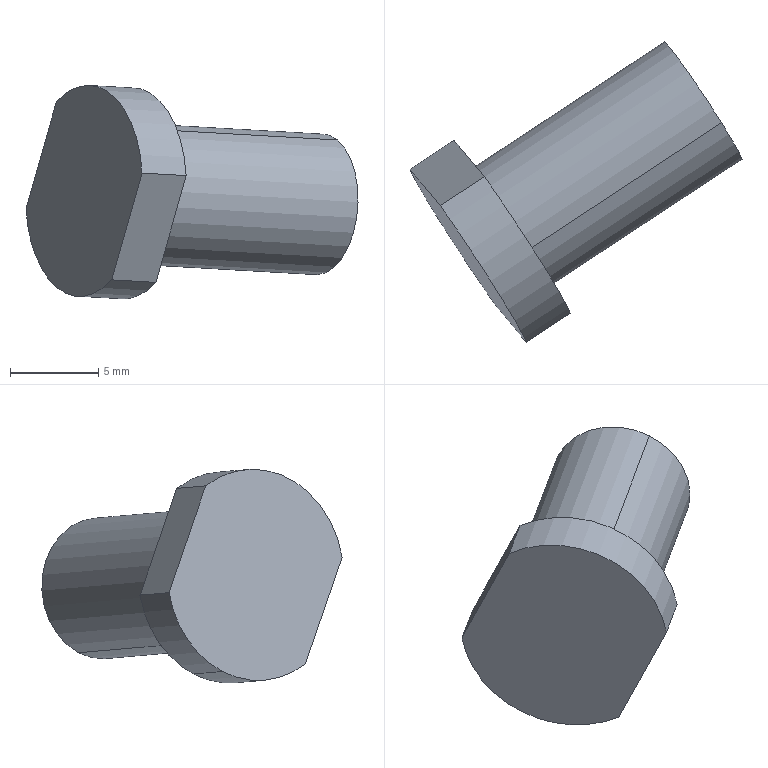Component | SolidWorks | KnucklePin-1 | 1 solid | 14 faces | box 18.85 x 17.05 x 12.13 mm | volume 788 mm3 | cylinder 7 | plane 5 | cone 2 | commonest cylinder face diameters 12 x3 4.2 x2 8 x2
build123d program:
from build123d import *

# Parameters (mm, degrees)
SKETCH1_R             = 6
BOSS_EXTRUDE1_DEPTH   = 3
SKETCH2_R             = 4
BOSS_EXTRUDE2_DEPTH   = 13
M5_TAPPED_HOLE1_D     = 4.2
M5_TAPPED_HOLE1_DEPTH = 12.4
M5_TAPPED_HOLE1_TIP   = 1.262
SKETCH4_W             = 12
SKETCH4_H             = 3
CUT_EXTRUDE1_DEPTH    = 1
SKETCH5_W             = 12
SKETCH5_H             = 3
CUT_EXTRUDE3_DEPTH    = 1


with BuildPart() as part:
    # Sketch1 → Boss-Extrude1 (new body)
    with BuildSketch(Plane.XY):
        Circle(SKETCH1_R)
    extrude(amount=BOSS_EXTRUDE1_DEPTH)

    # Sketch2 → Boss-Extrude2 (add)
    with BuildSketch(Plane(origin=(0, 0, 0), x_dir=(-1, 0, 0), z_dir=(0, 0, -1))):
        with Locations(Location((0, 0, 0), (0, 0, 180))):
            Circle(SKETCH2_R)
    extrude(amount=BOSS_EXTRUDE2_DEPTH)

    # M5 Tapped Hole1
    with Locations(Plane(origin=(0, 0, -13), x_dir=(-1, 0, 0), z_dir=(0, 0, -1))):
        with Locations((0, 0)):
            Hole(M5_TAPPED_HOLE1_D / 2, depth=M5_TAPPED_HOLE1_DEPTH)
            with Locations((0, 0, -(M5_TAPPED_HOLE1_DEPTH + M5_TAPPED_HOLE1_TIP / 2))):  # 118° drill point
                Cone(0, M5_TAPPED_HOLE1_D / 2, M5_TAPPED_HOLE1_TIP, mode=Mode.SUBTRACT)

    # Sketch4 → Cut-Extrude1 (cut)
    with BuildSketch(Plane(origin=(0, 6, 0), x_dir=(1, 0, 0), z_dir=(0, 1, 0))):
        with Locations((0, -1.5)):
            Rectangle(SKETCH4_W, SKETCH4_H)
    extrude(amount=-CUT_EXTRUDE1_DEPTH, mode=Mode.SUBTRACT)

    # Sketch5 → Cut-Extrude3 (cut)
    with BuildSketch(Plane(origin=(0, -6, 0), x_dir=(1, 0, 0), z_dir=(0, 1, 0))):
        with Locations((0, -1.5)):
            Rectangle(SKETCH5_W, SKETCH5_H)
    extrude(amount=CUT_EXTRUDE3_DEPTH, mode=Mode.SUBTRACT)


solid = part.part

# Placed as in the assembly
solid = solid.moved(Location((-123.505, 147.729, 689.195), (85.021, -56.519, 61.98)))
STEP:
#1=COLOUR_RGB('',0.7922,0.8196,0.9333);
#2=FILL_AREA_STYLE_COLOUR('',#1);
#3=FILL_AREA_STYLE('',(#2));
#4=SURFACE_STYLE_FILL_AREA(#3);
#5=SURFACE_SIDE_STYLE('',(#4));
#6=SURFACE_STYLE_USAGE(.BOTH.,#5);
#7=PRESENTATION_STYLE_ASSIGNMENT((#6));
#8=CARTESIAN_POINT('',(-4.821,5.803,27.208));
#9=VERTEX_POINT('',#8);
#10=CARTESIAN_POINT('',(-4.864,5.855,27.057));
#11=VERTEX_POINT('',#10);
#12=CARTESIAN_POINT('',(-4.843,5.829,27.133));
#13=DIRECTION('',(0.8341,0.5496,-0.04788));
#14=DIRECTION('',(-0.2592,0.3137,-0.9135));
#15=AXIS2_PLACEMENT_3D('',#12,#13,#14);
#16=CIRCLE('',#15,0.08268);
#17=EDGE_CURVE('',#9,#11,#16,.T.);
#18=ORIENTED_EDGE('',*,*,#17,.F.);
#19=CARTESIAN_POINT('',(-4.414,6.071,27.185));
#20=VERTEX_POINT('',#19);
#21=CARTESIAN_POINT('',(-4.414,6.071,27.185));
#22=DIRECTION('',(0.8341,0.5496,-0.04788));
#23=VECTOR('',#22,39.37);
#24=LINE('',#21,#23);
#25=EDGE_CURVE('',#9,#20,#24,.T.);
#26=ORIENTED_EDGE('',*,*,#25,.T.);
#27=CARTESIAN_POINT('',(-4.457,6.123,27.034));
#28=VERTEX_POINT('',#27);
#29=CARTESIAN_POINT('',(-4.436,6.097,27.109));
#30=DIRECTION('',(0.8341,0.5496,-0.04788));
#31=DIRECTION('',(-0.2592,0.3137,-0.9135));
#32=AXIS2_PLACEMENT_3D('',#29,#30,#31);
#33=CIRCLE('',#32,0.08268);
#34=EDGE_CURVE('',#20,#28,#33,.T.);
#35=ORIENTED_EDGE('',*,*,#34,.T.);
#36=CARTESIAN_POINT('',(-4.457,6.123,27.034));
#37=DIRECTION('',(0.8341,0.5496,-0.04788));
#38=VECTOR('',#37,39.37);
#39=LINE('',#36,#38);
#40=EDGE_CURVE('',#11,#28,#39,.T.);
#41=ORIENTED_EDGE('',*,*,#40,.F.);
#42=EDGE_LOOP('',(#18,#26,#35,#41));
#43=FACE_OUTER_BOUND('',#42,.T.);
#44=CARTESIAN_POINT('',(-4.436,6.097,27.109));
#45=DIRECTION('',(0.8341,0.5496,-0.04788));
#46=DIRECTION('',(-0.2592,0.3137,-0.9135));
#47=AXIS2_PLACEMENT_3D('',#44,#45,#46);
#48=CYLINDRICAL_SURFACE('',#47,0.08268);
#49=ADVANCED_FACE('',(#43),#48,.F.);
#50=CARTESIAN_POINT('',(-4.884,5.802,27.135));
#51=VERTEX_POINT('',#50);
#52=CARTESIAN_POINT('',(-4.864,5.855,27.057));
#53=DIRECTION('',(0.2074,0.552,-0.8076));
#54=VECTOR('',#53,39.37);
#55=LINE('',#52,#54);
#56=EDGE_CURVE('',#51,#11,#55,.T.);
#57=ORIENTED_EDGE('',*,*,#56,.F.);
#58=CARTESIAN_POINT('',(-4.821,5.803,27.208));
#59=DIRECTION('',(0.6517,0.01413,0.7583));
#60=VECTOR('',#59,39.37);
#61=LINE('',#58,#60);
#62=EDGE_CURVE('',#51,#9,#61,.T.);
#63=ORIENTED_EDGE('',*,*,#62,.T.);
#64=ORIENTED_EDGE('',*,*,#17,.T.);
#65=EDGE_LOOP('',(#57,#63,#64));
#66=FACE_OUTER_BOUND('',#65,.T.);
#67=CARTESIAN_POINT('',(-4.843,5.829,27.133));
#68=DIRECTION('',(0.8341,0.5496,-0.04788));
#69=DIRECTION('',(-0.2592,0.3137,-0.9135));
#70=AXIS2_PLACEMENT_3D('',#67,#68,#69);
#71=CONICAL_SURFACE('',#70,0.08268,1.03);
#72=ADVANCED_FACE('',(#66),#71,.F.);
#73=CARTESIAN_POINT('',(-4.476,6.147,26.965));
#74=VERTEX_POINT('',#73);
#75=CARTESIAN_POINT('',(-4.395,6.048,27.253));
#76=VERTEX_POINT('',#75);
#77=CARTESIAN_POINT('',(-4.436,6.097,27.109));
#78=DIRECTION('',(0.8341,0.5496,-0.04788));
#79=DIRECTION('',(-0.2592,0.3137,-0.9135));
#80=AXIS2_PLACEMENT_3D('',#77,#78,#79);
#81=CIRCLE('',#80,0.1575);
#82=EDGE_CURVE('',#74,#76,#81,.T.);
#83=ORIENTED_EDGE('',*,*,#82,.F.);
#84=CARTESIAN_POINT('',(-4.903,5.865,26.99));
#85=VERTEX_POINT('',#84);
#86=CARTESIAN_POINT('',(-4.476,6.147,26.965));
#87=DIRECTION('',(-0.8341,-0.5496,0.04788));
#88=VECTOR('',#87,39.37);
#89=LINE('',#86,#88);
#90=EDGE_CURVE('',#74,#85,#89,.T.);
#91=ORIENTED_EDGE('',*,*,#90,.T.);
#92=CARTESIAN_POINT('',(-4.822,5.767,27.278));
#93=VERTEX_POINT('',#92);
#94=CARTESIAN_POINT('',(-4.862,5.816,27.134));
#95=DIRECTION('',(0.8341,0.5496,-0.04788));
#96=DIRECTION('',(0.2592,-0.3137,0.9135));
#97=AXIS2_PLACEMENT_3D('',#94,#95,#96);
#98=CIRCLE('',#97,0.1575);
#99=EDGE_CURVE('',#85,#93,#98,.T.);
#100=ORIENTED_EDGE('',*,*,#99,.T.);
#101=CARTESIAN_POINT('',(-4.395,6.048,27.253));
#102=DIRECTION('',(-0.8341,-0.5496,0.04788));
#103=VECTOR('',#102,39.37);
#104=LINE('',#101,#103);
#105=EDGE_CURVE('',#76,#93,#104,.T.);
#106=ORIENTED_EDGE('',*,*,#105,.F.);
#107=EDGE_LOOP('',(#83,#91,#100,#106));
#108=FACE_OUTER_BOUND('',#107,.T.);
#109=CARTESIAN_POINT('',(-4.436,6.097,27.109));
#110=DIRECTION('',(-0.8341,-0.5496,0.04788));
#111=DIRECTION('',(0.2592,-0.3137,0.9135));
#112=AXIS2_PLACEMENT_3D('',#109,#110,#111);
#113=CYLINDRICAL_SURFACE('',#112,0.1575);
#114=ADVANCED_FACE('',(#108),#113,.T.);
#115=CARTESIAN_POINT('',(-5.022,5.825,26.924));
#116=VERTEX_POINT('',#115);
#117=CARTESIAN_POINT('',(-4.899,5.64,26.941));
#118=VERTEX_POINT('',#117);
#119=CARTESIAN_POINT('',(-4.961,5.751,27.139));
#120=DIRECTION('',(-0.8341,-0.5496,0.04788));
#121=DIRECTION('',(0.2592,-0.3137,0.9135));
#122=AXIS2_PLACEMENT_3D('',#119,#120,#121);
#123=CIRCLE('',#122,0.2362);
#124=EDGE_CURVE('',#116,#118,#123,.T.);
#125=ORIENTED_EDGE('',*,*,#124,.F.);
#126=CARTESIAN_POINT('',(-4.924,5.89,26.918));
#127=VERTEX_POINT('',#126);
#128=CARTESIAN_POINT('',(-5.022,5.825,26.924));
#129=DIRECTION('',(0.8341,0.5496,-0.04788));
#130=VECTOR('',#129,39.37);
#131=LINE('',#128,#130);
#132=EDGE_CURVE('',#116,#127,#131,.T.);
#133=ORIENTED_EDGE('',*,*,#132,.T.);
#134=CARTESIAN_POINT('',(-4.8,5.705,26.935));
#135=VERTEX_POINT('',#134);
#136=CARTESIAN_POINT('',(-4.862,5.816,27.134));
#137=DIRECTION('',(-0.8341,-0.5496,0.04788));
#138=DIRECTION('',(0.2592,-0.3137,0.9135));
#139=AXIS2_PLACEMENT_3D('',#136,#137,#138);
#140=CIRCLE('',#139,0.2362);
#141=EDGE_CURVE('',#127,#135,#140,.T.);
#142=ORIENTED_EDGE('',*,*,#141,.T.);
#143=CARTESIAN_POINT('',(-4.899,5.64,26.941));
#144=DIRECTION('',(-0.8341,-0.5496,0.04788));
#145=VECTOR('',#144,39.37);
#146=LINE('',#143,#145);
#147=EDGE_CURVE('',#135,#118,#146,.T.);
#148=ORIENTED_EDGE('',*,*,#147,.T.);
#149=EDGE_LOOP('',(#125,#133,#142,#148));
#150=FACE_OUTER_BOUND('',#149,.T.);
#151=CARTESIAN_POINT('',(-4.961,5.751,27.139));
#152=DIRECTION('',(0.8341,0.5496,-0.04788));
#153=DIRECTION('',(-0.2592,0.3137,-0.9135));
#154=AXIS2_PLACEMENT_3D('',#151,#152,#153);
#155=CYLINDRICAL_SURFACE('',#154,0.2362);
#156=ADVANCED_FACE('',(#150),#155,.T.);
#157=ORIENTED_EDGE('',*,*,#132,.F.);
#158=CARTESIAN_POINT('',(-5.091,5.945,27.1));
#159=VERTEX_POINT('',#158);
#160=CARTESIAN_POINT('',(-4.961,5.751,27.139));
#161=DIRECTION('',(-0.8341,-0.5496,0.04788));
#162=DIRECTION('',(0.2592,-0.3137,0.9135));
#163=AXIS2_PLACEMENT_3D('',#160,#161,#162);
#164=CIRCLE('',#163,0.2362);
#165=EDGE_CURVE('',#159,#116,#164,.T.);
#166=ORIENTED_EDGE('',*,*,#165,.F.);
#167=CARTESIAN_POINT('',(-4.992,6.009,27.094));
#168=VERTEX_POINT('',#167);
#169=CARTESIAN_POINT('',(-5.091,5.945,27.1));
#170=DIRECTION('',(-0.8341,-0.5496,0.04788));
#171=VECTOR('',#170,39.37);
#172=LINE('',#169,#171);
#173=EDGE_CURVE('',#168,#159,#172,.T.);
#174=ORIENTED_EDGE('',*,*,#173,.F.);
#175=CARTESIAN_POINT('',(-4.862,5.816,27.134));
#176=DIRECTION('',(-0.8341,-0.5496,0.04788));
#177=DIRECTION('',(0.2592,-0.3137,0.9135));
#178=AXIS2_PLACEMENT_3D('',#175,#176,#177);
#179=CIRCLE('',#178,0.2362);
#180=EDGE_CURVE('',#168,#127,#179,.T.);
#181=ORIENTED_EDGE('',*,*,#180,.T.);
#182=EDGE_LOOP('',(#157,#166,#174,#181));
#183=FACE_OUTER_BOUND('',#182,.T.);
#184=CARTESIAN_POINT('',(-4.961,5.751,27.139));
#185=DIRECTION('',(0.8341,0.5496,-0.04788));
#186=DIRECTION('',(-0.2592,0.3137,-0.9135));
#187=AXIS2_PLACEMENT_3D('',#184,#185,#186);
#188=CYLINDRICAL_SURFACE('',#187,0.2362);
#189=ADVANCED_FACE('',(#183),#188,.T.);
#190=CARTESIAN_POINT('',(-4.862,5.816,27.134));
#191=DIRECTION('',(0.8341,0.5496,-0.04788));
#192=DIRECTION('',(0.2592,-0.3137,0.9135));
#193=AXIS2_PLACEMENT_3D('',#190,#191,#192);
#194=CIRCLE('',#193,0.1575);
#195=EDGE_CURVE('',#93,#85,#194,.T.);
#196=ORIENTED_EDGE('',*,*,#195,.F.);
#197=ORIENTED_EDGE('',*,*,#99,.F.);
#198=EDGE_LOOP('',(#196,#197));
#199=FACE_BOUND('',#198,.T.);
#200=CARTESIAN_POINT('',(-4.733,5.623,27.173));
#201=VERTEX_POINT('',#200);
#202=CARTESIAN_POINT('',(-4.924,5.928,27.332));
#203=VERTEX_POINT('',#202);
#204=CARTESIAN_POINT('',(-4.862,5.816,27.134));
#205=DIRECTION('',(-0.8341,-0.5496,0.04788));
#206=DIRECTION('',(0.2592,-0.3137,0.9135));
#207=AXIS2_PLACEMENT_3D('',#204,#205,#206);
#208=CIRCLE('',#207,0.2362);
#209=EDGE_CURVE('',#201,#203,#208,.T.);
#210=ORIENTED_EDGE('',*,*,#209,.F.);
#211=CARTESIAN_POINT('',(-4.828,5.738,26.838));
#212=DIRECTION('',(-0.2592,0.3137,-0.9135));
#213=VECTOR('',#212,39.37);
#214=LINE('',#211,#213);
#215=EDGE_CURVE('',#201,#135,#214,.T.);
#216=ORIENTED_EDGE('',*,*,#215,.T.);
#217=ORIENTED_EDGE('',*,*,#141,.F.);
#218=ORIENTED_EDGE('',*,*,#180,.F.);
#219=CARTESIAN_POINT('',(-5.019,6.043,26.997));
#220=DIRECTION('',(-0.2592,0.3137,-0.9135));
#221=VECTOR('',#220,39.37);
#222=LINE('',#219,#221);
#223=EDGE_CURVE('',#203,#168,#222,.T.);
#224=ORIENTED_EDGE('',*,*,#223,.F.);
#225=EDGE_LOOP('',(#210,#216,#217,#218,#224));
#226=FACE_OUTER_BOUND('',#225,.T.);
#227=CARTESIAN_POINT('',(-4.862,5.816,27.134));
#228=DIRECTION('',(-0.8341,-0.5496,0.04788));
#229=DIRECTION('',(0.2592,-0.3137,0.9135));
#230=AXIS2_PLACEMENT_3D('',#227,#228,#229);
#231=PLANE('',#230);
#232=ADVANCED_FACE('',(#199,#226),#231,.F.);
#233=CARTESIAN_POINT('',(-4.831,5.558,27.179));
#234=VERTEX_POINT('',#233);
#235=CARTESIAN_POINT('',(-5.023,5.863,27.338));
#236=VERTEX_POINT('',#235);
#237=CARTESIAN_POINT('',(-4.961,5.751,27.139));
#238=DIRECTION('',(-0.8341,-0.5496,0.04788));
#239=DIRECTION('',(0.2592,-0.3137,0.9135));
#240=AXIS2_PLACEMENT_3D('',#237,#238,#239);
#241=CIRCLE('',#240,0.2362);
#242=EDGE_CURVE('',#234,#236,#241,.T.);
#243=ORIENTED_EDGE('',*,*,#242,.F.);
#244=CARTESIAN_POINT('',(-4.831,5.558,27.179));
#245=DIRECTION('',(0.8341,0.5496,-0.04788));
#246=VECTOR('',#245,39.37);
#247=LINE('',#244,#246);
#248=EDGE_CURVE('',#234,#201,#247,.T.);
#249=ORIENTED_EDGE('',*,*,#248,.T.);
#250=ORIENTED_EDGE('',*,*,#209,.T.);
#251=CARTESIAN_POINT('',(-5.023,5.863,27.338));
#252=DIRECTION('',(0.8341,0.5496,-0.04788));
#253=VECTOR('',#252,39.37);
#254=LINE('',#251,#253);
#255=EDGE_CURVE('',#236,#203,#254,.T.);
#256=ORIENTED_EDGE('',*,*,#255,.F.);
#257=EDGE_LOOP('',(#243,#249,#250,#256));
#258=FACE_OUTER_BOUND('',#257,.T.);
#259=CARTESIAN_POINT('',(-4.961,5.751,27.139));
#260=DIRECTION('',(0.8341,0.5496,-0.04788));
#261=DIRECTION('',(-0.2592,0.3137,-0.9135));
#262=AXIS2_PLACEMENT_3D('',#259,#260,#261);
#263=CYLINDRICAL_SURFACE('',#262,0.2362);
#264=ADVANCED_FACE('',(#258),#263,.T.);
#265=CARTESIAN_POINT('',(-4.865,5.599,27.06));
#266=DIRECTION('',(-0.2592,0.3137,-0.9135));
#267=VECTOR('',#266,39.37);
#268=LINE('',#265,#267);
#269=EDGE_CURVE('',#234,#118,#268,.T.);
#270=ORIENTED_EDGE('',*,*,#269,.F.);
#271=ORIENTED_EDGE('',*,*,#242,.T.);
#272=CARTESIAN_POINT('',(-5.057,5.904,27.219));
#273=DIRECTION('',(-0.2592,0.3137,-0.9135));
#274=VECTOR('',#273,39.37);
#275=LINE('',#272,#274);
#276=EDGE_CURVE('',#236,#159,#275,.T.);
#277=ORIENTED_EDGE('',*,*,#276,.T.);
#278=ORIENTED_EDGE('',*,*,#165,.T.);
#279=ORIENTED_EDGE('',*,*,#124,.T.);
#280=EDGE_LOOP('',(#270,#271,#277,#278,#279));
#281=FACE_OUTER_BOUND('',#280,.T.);
#282=CARTESIAN_POINT('',(-4.961,5.751,27.139));
#283=DIRECTION('',(-0.8341,-0.5496,0.04788));
#284=DIRECTION('',(0.2592,-0.3137,0.9135));
#285=AXIS2_PLACEMENT_3D('',#282,#283,#284);
#286=PLANE('',#285);
#287=ADVANCED_FACE('',(#281),#286,.T.);
#288=ORIENTED_EDGE('',*,*,#90,.F.);
#289=CARTESIAN_POINT('',(-4.436,6.097,27.109));
#290=DIRECTION('',(0.8341,0.5496,-0.04788));
#291=DIRECTION('',(-0.2592,0.3137,-0.9135));
#292=AXIS2_PLACEMENT_3D('',#289,#290,#291);
#293=CIRCLE('',#292,0.1575);
#294=EDGE_CURVE('',#76,#74,#293,.T.);
#295=ORIENTED_EDGE('',*,*,#294,.F.);
#296=ORIENTED_EDGE('',*,*,#105,.T.);
#297=ORIENTED_EDGE('',*,*,#195,.T.);
#298=EDGE_LOOP('',(#288,#295,#296,#297));
#299=FACE_OUTER_BOUND('',#298,.T.);
#300=CARTESIAN_POINT('',(-4.436,6.097,27.109));
#301=DIRECTION('',(-0.8341,-0.5496,0.04788));
#302=DIRECTION('',(0.2592,-0.3137,0.9135));
#303=AXIS2_PLACEMENT_3D('',#300,#301,#302);
#304=CYLINDRICAL_SURFACE('',#303,0.1575);
#305=ADVANCED_FACE('',(#299),#304,.T.);
#306=CARTESIAN_POINT('',(-4.436,6.097,27.109));
#307=DIRECTION('',(0.8341,0.5496,-0.04788));
#308=DIRECTION('',(-0.2592,0.3137,-0.9135));
#309=AXIS2_PLACEMENT_3D('',#306,#307,#308);
#310=CIRCLE('',#309,0.08268);
#311=EDGE_CURVE('',#28,#20,#310,.T.);
#312=ORIENTED_EDGE('',*,*,#311,.F.);
#313=ORIENTED_EDGE('',*,*,#34,.F.);
#314=EDGE_LOOP('',(#312,#313));
#315=FACE_BOUND('',#314,.T.);
#316=ORIENTED_EDGE('',*,*,#294,.T.);
#317=ORIENTED_EDGE('',*,*,#82,.T.);
#318=EDGE_LOOP('',(#316,#317));
#319=FACE_OUTER_BOUND('',#318,.T.);
#320=CARTESIAN_POINT('',(-4.436,6.097,27.109));
#321=DIRECTION('',(0.8341,0.5496,-0.04788));
#322=DIRECTION('',(-0.2592,0.3137,-0.9135));
#323=AXIS2_PLACEMENT_3D('',#320,#321,#322);
#324=PLANE('',#323);
#325=ADVANCED_FACE('',(#315,#319),#324,.T.);
#326=ORIENTED_EDGE('',*,*,#62,.F.);
#327=ORIENTED_EDGE('',*,*,#56,.T.);
#328=CARTESIAN_POINT('',(-4.843,5.829,27.133));
#329=DIRECTION('',(0.8341,0.5496,-0.04788));
#330=DIRECTION('',(-0.2592,0.3137,-0.9135));
#331=AXIS2_PLACEMENT_3D('',#328,#329,#330);
#332=CIRCLE('',#331,0.08268);
#333=EDGE_CURVE('',#11,#9,#332,.T.);
#334=ORIENTED_EDGE('',*,*,#333,.T.);
#335=EDGE_LOOP('',(#326,#327,#334));
#336=FACE_OUTER_BOUND('',#335,.T.);
#337=CARTESIAN_POINT('',(-4.843,5.829,27.133));
#338=DIRECTION('',(0.8341,0.5496,-0.04788));
#339=DIRECTION('',(-0.2592,0.3137,-0.9135));
#340=AXIS2_PLACEMENT_3D('',#337,#338,#339);
#341=CONICAL_SURFACE('',#340,0.08268,1.03);
#342=ADVANCED_FACE('',(#336),#341,.F.);
#343=ORIENTED_EDGE('',*,*,#25,.F.);
#344=ORIENTED_EDGE('',*,*,#333,.F.);
#345=ORIENTED_EDGE('',*,*,#40,.T.);
#346=ORIENTED_EDGE('',*,*,#311,.T.);
#347=EDGE_LOOP('',(#343,#344,#345,#346));
#348=FACE_OUTER_BOUND('',#347,.T.);
#349=CARTESIAN_POINT('',(-4.436,6.097,27.109));
#350=DIRECTION('',(0.8341,0.5496,-0.04788));
#351=DIRECTION('',(-0.2592,0.3137,-0.9135));
#352=AXIS2_PLACEMENT_3D('',#349,#350,#351);
#353=CYLINDRICAL_SURFACE('',#352,0.08268);
#354=ADVANCED_FACE('',(#348),#353,.F.);
#355=ORIENTED_EDGE('',*,*,#255,.T.);
#356=ORIENTED_EDGE('',*,*,#223,.T.);
#357=ORIENTED_EDGE('',*,*,#173,.T.);
#358=ORIENTED_EDGE('',*,*,#276,.F.);
#359=EDGE_LOOP('',(#355,#356,#357,#358));
#360=FACE_OUTER_BOUND('',#359,.T.);
#361=CARTESIAN_POINT('',(-4.958,5.969,27.213));
#362=DIRECTION('',(-0.487,0.7743,0.4041));
#363=DIRECTION('',(-0.8341,-0.5496,0.04788));
#364=AXIS2_PLACEMENT_3D('',#361,#362,#363);
#365=PLANE('',#364);
#366=ADVANCED_FACE('',(#360),#365,.T.);
#367=ORIENTED_EDGE('',*,*,#269,.T.);
#368=ORIENTED_EDGE('',*,*,#147,.F.);
#369=ORIENTED_EDGE('',*,*,#215,.F.);
#370=ORIENTED_EDGE('',*,*,#248,.F.);
#371=EDGE_LOOP('',(#367,#368,#369,#370));
#372=FACE_OUTER_BOUND('',#371,.T.);
#373=CARTESIAN_POINT('',(-4.767,5.664,27.054));
#374=DIRECTION('',(-0.487,0.7743,0.4041));
#375=DIRECTION('',(-0.8341,-0.5496,0.04788));
#376=AXIS2_PLACEMENT_3D('',#373,#374,#375);
#377=PLANE('',#376);
#378=ADVANCED_FACE('',(#372),#377,.F.);
#379=CLOSED_SHELL('',(#49,#72,#114,#156,#189,#232,#264,#287,#305,#325,#342,#354,#366,#378));
#380=MANIFOLD_SOLID_BREP('',#379);
#381=STYLED_ITEM('',(#7),#380);
#382=(LENGTH_UNIT()NAMED_UNIT(*)SI_UNIT($,.METRE.));
#383=LENGTH_MEASURE_WITH_UNIT(LENGTH_MEASURE(0.0254),#382);
#384=DIMENSIONAL_EXPONENTS(1.,0.,0.,0.,0.,0.,0.);
#385=(CONVERSION_BASED_UNIT('',#383)LENGTH_UNIT()NAMED_UNIT(#384));
#386=UNCERTAINTY_MEASURE_WITH_UNIT(LENGTH_MEASURE(0.00001),#385,'','');
#387=(NAMED_UNIT(*)PLANE_ANGLE_UNIT()SI_UNIT($,.RADIAN.));
#388=(NAMED_UNIT(*)SI_UNIT($,.STERADIAN.)SOLID_ANGLE_UNIT());
#389=(GEOMETRIC_REPRESENTATION_CONTEXT(3)GLOBAL_UNCERTAINTY_ASSIGNED_CONTEXT((#386))GLOBAL_UNIT_ASSIGNED_CONTEXT((#385,#387,#388))REPRESENTATION_CONTEXT('',''));
#390=MECHANICAL_DESIGN_GEOMETRIC_PRESENTATION_REPRESENTATION('',(#381),#389);
#391=CARTESIAN_POINT('',(0.,0.,0.));
#392=DIRECTION('',(0.,0.,1.));
#393=DIRECTION('',(1.,0.,0.));
#394=AXIS2_PLACEMENT_3D('',#391,#392,#393);
#395=(LENGTH_UNIT()NAMED_UNIT(*)SI_UNIT($,.METRE.));
#396=LENGTH_MEASURE_WITH_UNIT(LENGTH_MEASURE(0.0254),#395);
#397=DIMENSIONAL_EXPONENTS(1.,0.,0.,0.,0.,0.,0.);
#398=(CONVERSION_BASED_UNIT('',#396)LENGTH_UNIT()NAMED_UNIT(#397));
#399=UNCERTAINTY_MEASURE_WITH_UNIT(LENGTH_MEASURE(0.00001),#398,'','');
#400=(NAMED_UNIT(*)PLANE_ANGLE_UNIT()SI_UNIT($,.RADIAN.));
#401=(NAMED_UNIT(*)SI_UNIT($,.STERADIAN.)SOLID_ANGLE_UNIT());
#402=(GEOMETRIC_REPRESENTATION_CONTEXT(3)GLOBAL_UNCERTAINTY_ASSIGNED_CONTEXT((#399))GLOBAL_UNIT_ASSIGNED_CONTEXT((#398,#400,#401))REPRESENTATION_CONTEXT('',''));
#403=ADVANCED_BREP_SHAPE_REPRESENTATION('',(#380,#394),#402);
#404=PRESENTATION_LAYER_ASSIGNMENT('','',(#381));